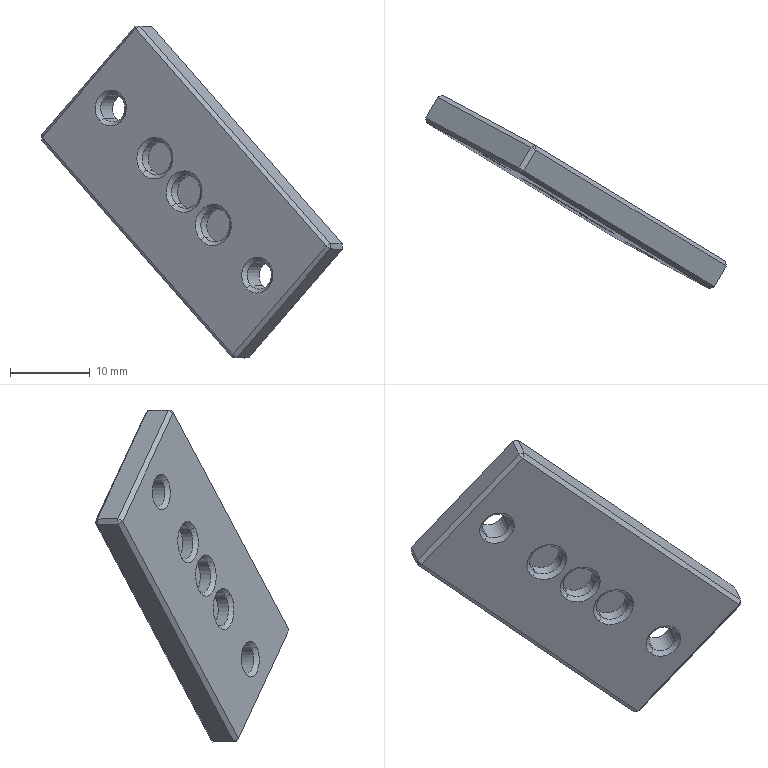Component | SolidWorks | 5z0-123-1 | 1 solid | 53 faces | box 37.65 x 24.27 x 41.61 mm | volume 2997 mm3 | plane 29 | cone 14 | cylinder 10 | commonest cylinder face diameters 4.2 x6 3.5 x4
build123d program:
from build123d import *

# Parameters (mm, degrees)
SKETCH1_W           = 20
SKETCH1_H           = 40
BOSS_EXTRUDE1_DEPTH = 4
SKETCH3_R           = 1.75
CUT_EXTRUDE2_DEPTH  = 23.716
SKETCH4_R           = 2.1
CUT_EXTRUDE3_DEPTH  = 2
LPATTERN1_COUNT     = 2
LPATTERN1_PITCH     = 6
LPATTERN2_COUNT     = 2
LPATTERN2_PITCH     = 6
CHAMFER1_SIZE       = 0.5


with BuildPart() as part:
    # Sketch1 → Boss-Extrude1 (new body)
    with BuildSketch(Plane.XY):
        Rectangle(SKETCH1_W, SKETCH1_H)
    extrude(amount=BOSS_EXTRUDE1_DEPTH)

    # Sketch3 → Cut-Extrude2 (cut, through all)
    with BuildSketch(Plane.XY.offset(4)):
        with Locations((0, 15)):
            Circle(SKETCH3_R)
        with Locations((0, -15)):
            Circle(SKETCH3_R)
    extrude(amount=-CUT_EXTRUDE2_DEPTH, mode=Mode.SUBTRACT)

    # Sketch4 → Cut-Extrude3 (cut)
    with BuildSketch(Plane(origin=(0, 0, 0), x_dir=(-1, 0, 0), z_dir=(0, 0, -1))):
        Circle(SKETCH4_R)
    cut_extrude3 = extrude(amount=-CUT_EXTRUDE3_DEPTH, mode=Mode.SUBTRACT)

    # LPattern1: Cut-Extrude3 ×2
    with Locations(*[(0, -i * LPATTERN1_PITCH, 0) for i in range(1, LPATTERN1_COUNT)]):
        add(cut_extrude3, mode=Mode.SUBTRACT)

    # LPattern2: Cut-Extrude3 ×2
    with Locations(*[(0, i * LPATTERN2_PITCH, 0) for i in range(1, LPATTERN2_COUNT)]):
        add(cut_extrude3, mode=Mode.SUBTRACT)

    # Chamfer1
    chamfer1_edges = [part.edges().sort_by_distance(p)[0] for p in [
        (-10, 0, 4),
        (0, -20, 4),
        (-1.75, 15, 0),
        (-1.75, 15, 4),
        (-1.75, -15, 0),
        (-1.75, -15, 4),
        (2.1, 0, 0),
        (2.1, -6, 0),
        (2.1, 6, 0),
        (10, 0, 4),
        (0, -20, 0),
        (-10, 0, 0),
        (0, 20, 0),
        (10, 0, 0),
        (0, 20, 4),
        (10, -20, 2),
        (-10, -20, 2),
        (-10, 20, 2),
        (10, 20, 2),
    ]]
    chamfer(chamfer1_edges, length=CHAMFER1_SIZE)


solid = part.part

# Placed as in the assembly
solid = solid.moved(Location((-78.851, -91.285, 77.48), (-91.664, 29.849, 135.13)))